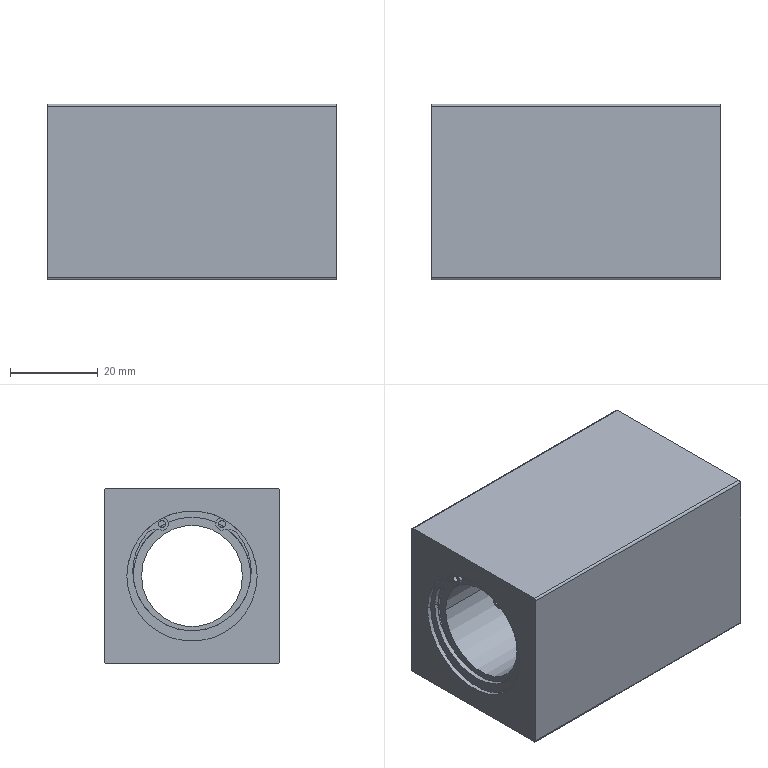Component | SolidWorks | RMS_20X400_03-1_RMS20X50_Body-1 | 1 solid | 100 faces | box 66 x 40 x 40 mm | volume 76860 mm3 | cylinder 54 | plane 30 | cone 16 | commonest cylinder face diameters 1.6 x8 2.5 x8 4 x8 27 x6 2.823 x6 26.81 x4 29.667 x4 1 x4
build123d program:
from build123d import *

# Parameters (mm, degrees)
SKETCH1_R           = 11.5
BOSS_EXTRUDE1_DEPTH = 66
BOSS_EXTRUDE2_START = -1
SKETCH8_R           = 0.8
BOSS_EXTRUDE2_DEPTH = 1
SKETCH9_R           = 0.8
BOSS_EXTRUDE3_DEPTH = 1


with BuildPart() as part:
    # Sketch1 → Boss-Extrude1 (new body)
    with BuildSketch(Plane(origin=(0, 0, 0), x_dir=(0, 0, -1), z_dir=(1, 0, 0))):
        with BuildLine():
            Line((-19.5, -20), (19.5, -20))
            ThreePointArc((19.5, -20), (19.854, -19.854), (20, -19.5))
            Line((20, -19.5), (20, 19.5))
            ThreePointArc((20, 19.5), (19.854, 19.854), (19.5, 20))
            Line((19.5, 20), (-19.5, 20))
            ThreePointArc((-19.5, 20), (-19.854, 19.854), (-20, 19.5))
            Line((-20, 19.5), (-20, -19.5))
            ThreePointArc((-20, -19.5), (-19.854, -19.854), (-19.5, -20))
        make_face()
        Circle(SKETCH1_R, mode=Mode.SUBTRACT)
    extrude(amount=BOSS_EXTRUDE1_DEPTH)

    # Sketch2 → Cut-Revolve1 (revolve, cut)
    with BuildSketch(Plane(origin=(58, 0, 0), x_dir=(0, 0, -1), z_dir=(1, 0, 0)), mode=Mode.PRIVATE) as cut_revolve1_sk:
        Polygon((-13.278, 12.5), (-14, 11.25), (-14.5, 11.25), (-14.5, 10.5), (-19.57, 10.5), (-20, 10.07), (-20, 12.5), align=None)
    revolve(cut_revolve1_sk.sketch.rotate(Axis((58, 12.5, 20), (0, 0, -1)), 90), axis=Axis((58, 12.5, 20), (0, 0, -1)), mode=Mode.SUBTRACT)

    # Sketch3 → Cut-Revolve2 (revolve, cut)
    with BuildSketch(Plane(origin=(58, 0, 0), x_dir=(0, 0, -1), z_dir=(1, 0, 0)), mode=Mode.PRIVATE) as cut_revolve2_sk:
        Polygon((-20, -12.5), (-20, -10.07), (-19.57, -10.5), (-14.5, -10.5), (-14.5, -11.25), (-14, -11.25), (-13.278, -12.5), align=None)
    revolve(cut_revolve2_sk.sketch.rotate(Axis((58, -12.5, 13.278), (0, 0, 1)), 270), axis=Axis((58, -12.5, 13.278), (0, 0, 1)), mode=Mode.SUBTRACT)

    # Sketch4 → Cut-Revolve3 (revolve, cut)
    with BuildSketch(Plane(origin=(8, 0, 0), x_dir=(0, 0, -1), z_dir=(1, 0, 0)), mode=Mode.PRIVATE) as cut_revolve3_sk:
        Polygon((-13.278, 12.5), (-14, 11.25), (-14.5, 11.25), (-14.5, 10.5), (-19.57, 10.5), (-20, 10.07), (-20, 12.5), align=None)
    revolve(cut_revolve3_sk.sketch.rotate(Axis((8, 12.5, 20), (0, 0, -1)), 90), axis=Axis((8, 12.5, 20), (0, 0, -1)), mode=Mode.SUBTRACT)

    # Sketch5 → Cut-Revolve4 (revolve, cut)
    with BuildSketch(Plane(origin=(8, 0, 0), x_dir=(0, 0, -1), z_dir=(1, 0, 0)), mode=Mode.PRIVATE) as cut_revolve4_sk:
        Polygon((-20, -12.5), (-20, -10.07), (-19.57, -10.5), (-14.5, -10.5), (-14.5, -11.25), (-14, -11.25), (-13.278, -12.5), align=None)
    revolve(cut_revolve4_sk.sketch.rotate(Axis((8, -12.5, 13.278), (0, 0, 1)), 270), axis=Axis((8, -12.5, 13.278), (0, 0, 1)), mode=Mode.SUBTRACT)

    # Sketch6 → Cut-Revolve5 (revolve, cut)
    with BuildSketch(Plane.XY, mode=Mode.PRIVATE) as cut_revolve5_sk:
        Polygon((0, 11.5), (2.5, 11.5), (2.5, 13.405), (2, 13.405), (2, 14.833), (0, 14.833), align=None)
    revolve(cut_revolve5_sk.sketch.rotate(Axis((66, 0, 0), (-1, 0, 0)), 270), axis=Axis((66, 0, 0), (-1, 0, 0)), mode=Mode.SUBTRACT)

    # Sketch7 → Cut-Revolve6 (revolve, cut)
    with BuildSketch(Plane.XY, mode=Mode.PRIVATE) as cut_revolve6_sk:
        Polygon((63.5, 11.5), (66, 11.5), (66, 14.833), (64, 14.833), (64, 13.405), (63.5, 13.405), align=None)
    revolve(cut_revolve6_sk.sketch.rotate(Axis((66, 0, 0), (-1, 0, 0)), 270), axis=Axis((66, 0, 0), (-1, 0, 0)), mode=Mode.SUBTRACT)

    # Sketch8 → Boss-Extrude2 (add)
    with BuildSketch(Plane(origin=(2, 0, 0), x_dir=(0, 0, -1), z_dir=(1, 0, 0)).offset(BOSS_EXTRUDE2_START)):
        with BuildLine():
            ThreePointArc((6.689, -13.24), (0, 14.833), (-6.689, -13.24))
            ThreePointArc((-6.689, -13.24), (-5.49, -11.403), (-7.535, -10.611))
            ThreePointArc((-7.535, -10.611), (-9.126, -10.491), (-10.429, -9.572))
            ThreePointArc((-10.429, -9.572), (0, 12.5), (10.429, -9.572))
            ThreePointArc((10.429, -9.572), (9.126, -10.491), (7.535, -10.611))
            ThreePointArc((7.535, -10.611), (5.49, -11.403), (6.689, -13.24))
        make_face()
        with Locations((6.833, -11.836)):
            Circle(SKETCH8_R, mode=Mode.SUBTRACT)
        with Locations((-6.833, -11.836)):
            Circle(SKETCH8_R, mode=Mode.SUBTRACT)
    extrude(amount=BOSS_EXTRUDE2_DEPTH)

    # Sketch9 → Boss-Extrude3 (add)
    with BuildSketch(Plane(origin=(64, 0, 0), x_dir=(0, 0, -1), z_dir=(1, 0, 0))):
        with BuildLine():
            ThreePointArc((6.689, -13.24), (0, 14.833), (-6.689, -13.24))
            ThreePointArc((-6.689, -13.24), (-5.49, -11.403), (-7.535, -10.611))
            ThreePointArc((-7.535, -10.611), (-9.126, -10.491), (-10.429, -9.572))
            ThreePointArc((-10.429, -9.572), (0, 12.5), (10.429, -9.572))
            ThreePointArc((10.429, -9.572), (9.126, -10.491), (7.535, -10.611))
            ThreePointArc((7.535, -10.611), (5.49, -11.403), (6.689, -13.24))
        make_face()
        with Locations((6.833, -11.836)):
            Circle(SKETCH9_R, mode=Mode.SUBTRACT)
        with Locations((-6.833, -11.836)):
            Circle(SKETCH9_R, mode=Mode.SUBTRACT)
    extrude(amount=BOSS_EXTRUDE3_DEPTH)


solid = part.part

# Placed as in the assembly
solid = solid.moved(Location((-5.119, 21, 41.5), (-90, 0, 0)))